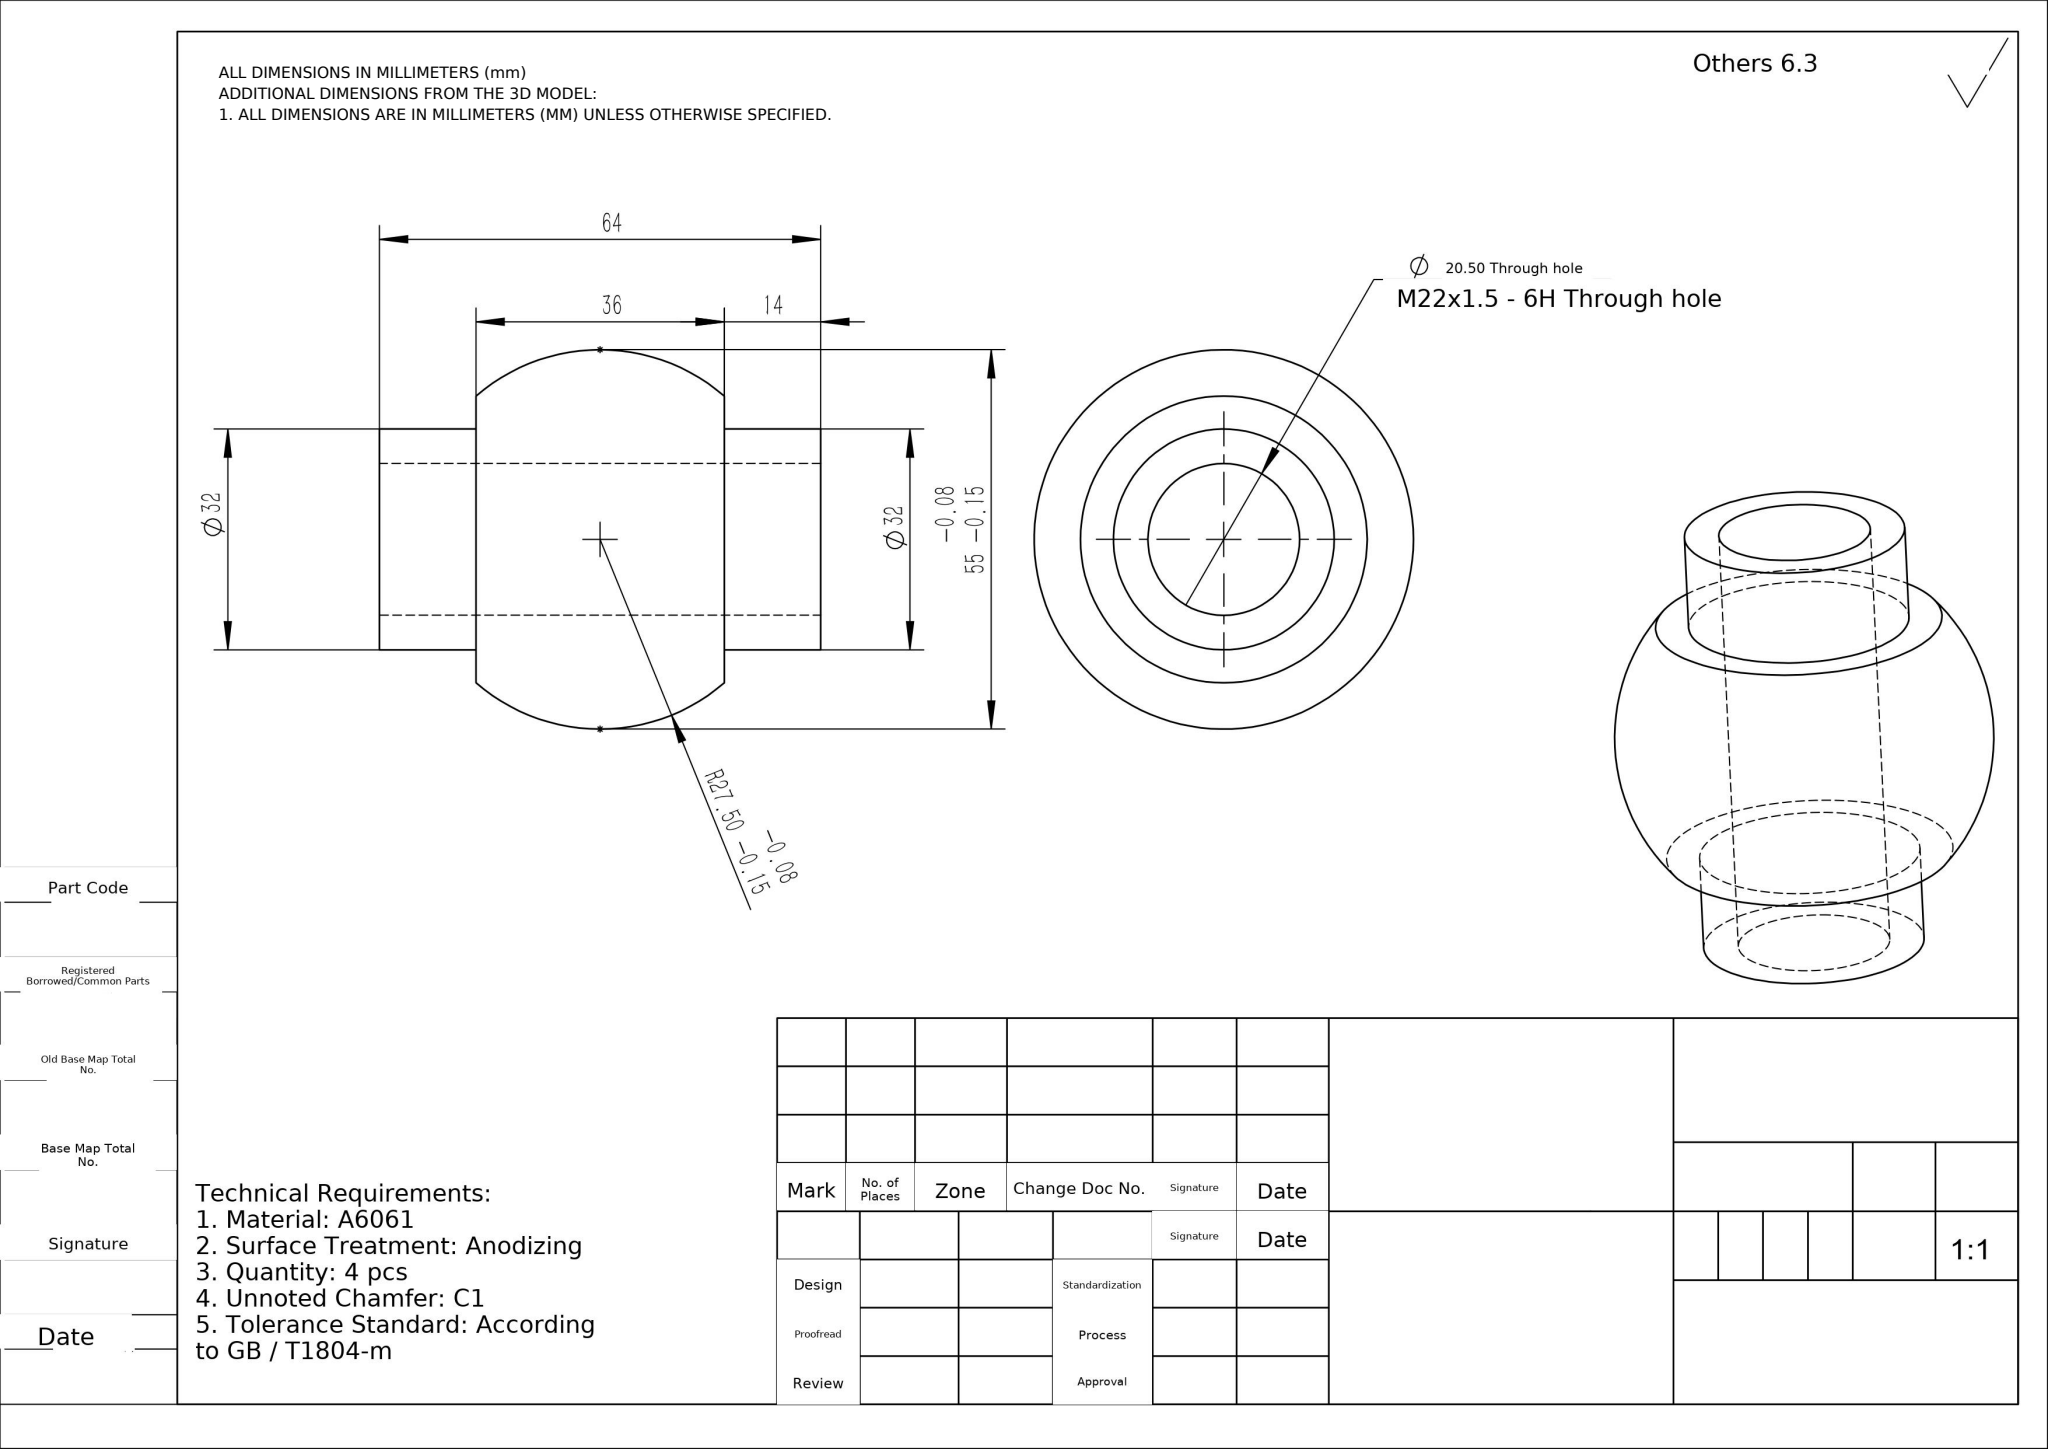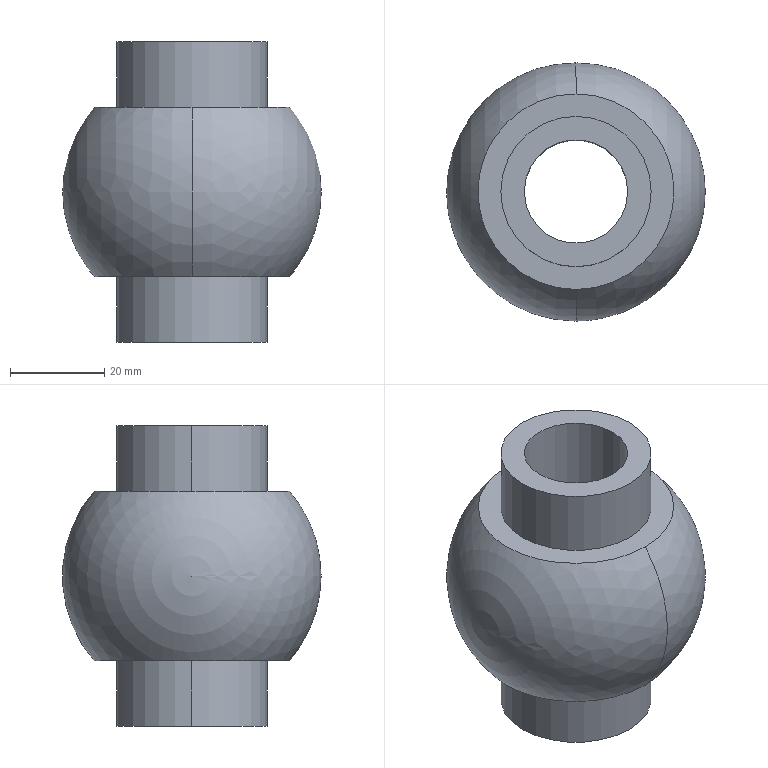Part | NX | mm | Spherical Flanged Bushing | 1 solid | 12 faces | box 55 x 55 x 64 mm | volume 71506 mm3 | cylinder 6 | plane 4 | sphere 2 | commonest cylinder face diameters 32 x4 22 x2
STEP:
#1=COLOUR_RGB('',0.,0.502,0.502);
#2=FILL_AREA_STYLE_COLOUR('',#1);
#3=FILL_AREA_STYLE('',(#2));
#4=SURFACE_STYLE_FILL_AREA(#3);
#5=SURFACE_SIDE_STYLE('',(#4));
#6=SURFACE_STYLE_USAGE(.BOTH.,#5);
#7=PRESENTATION_STYLE_ASSIGNMENT((#6));
#8=CARTESIAN_POINT('',(-11.,0.,-32.));
#9=VERTEX_POINT('',#8);
#10=CARTESIAN_POINT('',(11.,0.,-32.));
#11=VERTEX_POINT('',#10);
#12=CARTESIAN_POINT('',(0.,0.,-32.));
#13=DIRECTION('',(0.,0.,1.));
#14=DIRECTION('',(1.,0.,0.));
#15=AXIS2_PLACEMENT_3D('',#12,#13,#14);
#16=CIRCLE('',#15,11.);
#17=EDGE_CURVE('',#9,#11,#16,.T.);
#18=ORIENTED_EDGE('',*,*,#17,.F.);
#19=CARTESIAN_POINT('',(-11.,0.,32.));
#20=VERTEX_POINT('',#19);
#21=CARTESIAN_POINT('',(-11.,0.,32.));
#22=DIRECTION('',(0.,0.,1.));
#23=VECTOR('',#22,1000.);
#24=LINE('',#21,#23);
#25=EDGE_CURVE('',#9,#20,#24,.T.);
#26=ORIENTED_EDGE('',*,*,#25,.T.);
#27=CARTESIAN_POINT('',(11.,0.,32.));
#28=VERTEX_POINT('',#27);
#29=CARTESIAN_POINT('',(0.,0.,32.));
#30=DIRECTION('',(0.,0.,1.));
#31=DIRECTION('',(1.,0.,0.));
#32=AXIS2_PLACEMENT_3D('',#29,#30,#31);
#33=CIRCLE('',#32,11.);
#34=EDGE_CURVE('',#20,#28,#33,.T.);
#35=ORIENTED_EDGE('',*,*,#34,.T.);
#36=CARTESIAN_POINT('',(11.,0.,32.));
#37=DIRECTION('',(0.,0.,1.));
#38=VECTOR('',#37,1000.);
#39=LINE('',#36,#38);
#40=EDGE_CURVE('',#11,#28,#39,.T.);
#41=ORIENTED_EDGE('',*,*,#40,.F.);
#42=EDGE_LOOP('',(#18,#26,#35,#41));
#43=FACE_OUTER_BOUND('',#42,.T.);
#44=CARTESIAN_POINT('',(0.,0.,32.));
#45=DIRECTION('',(0.,0.,1.));
#46=DIRECTION('',(1.,0.,0.));
#47=AXIS2_PLACEMENT_3D('',#44,#45,#46);
#48=CYLINDRICAL_SURFACE('',#47,11.);
#49=ADVANCED_FACE('',(#43),#48,.F.);
#50=CARTESIAN_POINT('',(16.,0.,32.));
#51=VERTEX_POINT('',#50);
#52=CARTESIAN_POINT('',(-16.,0.,32.));
#53=VERTEX_POINT('',#52);
#54=CARTESIAN_POINT('',(0.,0.,32.));
#55=DIRECTION('',(0.,0.,1.));
#56=DIRECTION('',(1.,0.,0.));
#57=AXIS2_PLACEMENT_3D('',#54,#55,#56);
#58=CIRCLE('',#57,16.);
#59=EDGE_CURVE('',#51,#53,#58,.T.);
#60=ORIENTED_EDGE('',*,*,#59,.F.);
#61=CARTESIAN_POINT('',(16.,0.,18.));
#62=VERTEX_POINT('',#61);
#63=CARTESIAN_POINT('',(16.,0.,32.));
#64=DIRECTION('',(0.,0.,-1.));
#65=VECTOR('',#64,1000.);
#66=LINE('',#63,#65);
#67=EDGE_CURVE('',#51,#62,#66,.T.);
#68=ORIENTED_EDGE('',*,*,#67,.T.);
#69=CARTESIAN_POINT('',(-16.,0.,18.));
#70=VERTEX_POINT('',#69);
#71=CARTESIAN_POINT('',(0.,0.,18.));
#72=DIRECTION('',(0.,0.,-1.));
#73=DIRECTION('',(-1.,0.,0.));
#74=AXIS2_PLACEMENT_3D('',#71,#72,#73);
#75=CIRCLE('',#74,16.);
#76=EDGE_CURVE('',#70,#62,#75,.T.);
#77=ORIENTED_EDGE('',*,*,#76,.F.);
#78=CARTESIAN_POINT('',(-16.,0.,32.));
#79=DIRECTION('',(0.,0.,-1.));
#80=VECTOR('',#79,1000.);
#81=LINE('',#78,#80);
#82=EDGE_CURVE('',#53,#70,#81,.T.);
#83=ORIENTED_EDGE('',*,*,#82,.F.);
#84=EDGE_LOOP('',(#60,#68,#77,#83));
#85=FACE_OUTER_BOUND('',#84,.T.);
#86=CARTESIAN_POINT('',(0.,0.,32.));
#87=DIRECTION('',(0.,0.,-1.));
#88=DIRECTION('',(-1.,0.,0.));
#89=AXIS2_PLACEMENT_3D('',#86,#87,#88);
#90=CYLINDRICAL_SURFACE('',#89,16.);
#91=ADVANCED_FACE('',(#85),#90,.T.);
#92=CARTESIAN_POINT('',(0.,-20.791,18.));
#93=VERTEX_POINT('',#92);
#94=CARTESIAN_POINT('',(-0.,20.791,18.));
#95=VERTEX_POINT('',#94);
#96=CARTESIAN_POINT('',(0.,0.,18.));
#97=DIRECTION('',(0.,0.,-1.));
#98=DIRECTION('',(-1.,0.,0.));
#99=AXIS2_PLACEMENT_3D('',#96,#97,#98);
#100=CIRCLE('',#99,20.791);
#101=EDGE_CURVE('',#93,#95,#100,.T.);
#102=ORIENTED_EDGE('',*,*,#101,.T.);
#103=CARTESIAN_POINT('',(-0.,20.791,-18.));
#104=VERTEX_POINT('',#103);
#105=CARTESIAN_POINT('',(0.,0.,0.));
#106=DIRECTION('',(-1.,-0.,0.));
#107=DIRECTION('',(0.,-1.,0.));
#108=AXIS2_PLACEMENT_3D('',#105,#106,#107);
#109=CIRCLE('',#108,27.5);
#110=EDGE_CURVE('',#95,#104,#109,.T.);
#111=ORIENTED_EDGE('',*,*,#110,.T.);
#112=CARTESIAN_POINT('',(0.,-20.791,-18.));
#113=VERTEX_POINT('',#112);
#114=CARTESIAN_POINT('',(0.,0.,-18.));
#115=DIRECTION('',(0.,0.,-1.));
#116=DIRECTION('',(-1.,0.,0.));
#117=AXIS2_PLACEMENT_3D('',#114,#115,#116);
#118=CIRCLE('',#117,20.791);
#119=EDGE_CURVE('',#113,#104,#118,.T.);
#120=ORIENTED_EDGE('',*,*,#119,.F.);
#121=CARTESIAN_POINT('',(0.,0.,0.));
#122=DIRECTION('',(1.,0.,0.));
#123=DIRECTION('',(0.,0.,-1.));
#124=AXIS2_PLACEMENT_3D('',#121,#122,#123);
#125=CIRCLE('',#124,27.5);
#126=EDGE_CURVE('',#93,#113,#125,.T.);
#127=ORIENTED_EDGE('',*,*,#126,.F.);
#128=EDGE_LOOP('',(#102,#111,#120,#127));
#129=FACE_OUTER_BOUND('',#128,.T.);
#130=CARTESIAN_POINT('',(0.,0.,0.));
#131=DIRECTION('',(-1.,0.,0.));
#132=DIRECTION('',(0.,-1.,0.));
#133=AXIS2_PLACEMENT_3D('',#130,#131,#132);
#134=SPHERICAL_SURFACE('',#133,27.5);
#135=ADVANCED_FACE('',(#129),#134,.T.);
#136=CARTESIAN_POINT('',(16.,0.,-18.));
#137=VERTEX_POINT('',#136);
#138=CARTESIAN_POINT('',(-16.,0.,-18.));
#139=VERTEX_POINT('',#138);
#140=CARTESIAN_POINT('',(0.,0.,-18.));
#141=DIRECTION('',(0.,0.,1.));
#142=DIRECTION('',(1.,0.,0.));
#143=AXIS2_PLACEMENT_3D('',#140,#141,#142);
#144=CIRCLE('',#143,16.);
#145=EDGE_CURVE('',#137,#139,#144,.T.);
#146=ORIENTED_EDGE('',*,*,#145,.F.);
#147=CARTESIAN_POINT('',(16.,0.,-32.));
#148=VERTEX_POINT('',#147);
#149=CARTESIAN_POINT('',(16.,0.,32.));
#150=DIRECTION('',(0.,0.,-1.));
#151=VECTOR('',#150,1000.);
#152=LINE('',#149,#151);
#153=EDGE_CURVE('',#137,#148,#152,.T.);
#154=ORIENTED_EDGE('',*,*,#153,.T.);
#155=CARTESIAN_POINT('',(-16.,0.,-32.));
#156=VERTEX_POINT('',#155);
#157=CARTESIAN_POINT('',(0.,0.,-32.));
#158=DIRECTION('',(0.,0.,1.));
#159=DIRECTION('',(1.,0.,0.));
#160=AXIS2_PLACEMENT_3D('',#157,#158,#159);
#161=CIRCLE('',#160,16.);
#162=EDGE_CURVE('',#148,#156,#161,.T.);
#163=ORIENTED_EDGE('',*,*,#162,.T.);
#164=CARTESIAN_POINT('',(-16.,0.,32.));
#165=DIRECTION('',(0.,0.,-1.));
#166=VECTOR('',#165,1000.);
#167=LINE('',#164,#166);
#168=EDGE_CURVE('',#139,#156,#167,.T.);
#169=ORIENTED_EDGE('',*,*,#168,.F.);
#170=EDGE_LOOP('',(#146,#154,#163,#169));
#171=FACE_OUTER_BOUND('',#170,.T.);
#172=CARTESIAN_POINT('',(0.,0.,32.));
#173=DIRECTION('',(0.,0.,-1.));
#174=DIRECTION('',(-1.,0.,0.));
#175=AXIS2_PLACEMENT_3D('',#172,#173,#174);
#176=CYLINDRICAL_SURFACE('',#175,16.);
#177=ADVANCED_FACE('',(#171),#176,.T.);
#178=ORIENTED_EDGE('',*,*,#153,.F.);
#179=CARTESIAN_POINT('',(0.,0.,-18.));
#180=DIRECTION('',(0.,0.,1.));
#181=DIRECTION('',(1.,0.,0.));
#182=AXIS2_PLACEMENT_3D('',#179,#180,#181);
#183=CIRCLE('',#182,16.);
#184=EDGE_CURVE('',#139,#137,#183,.T.);
#185=ORIENTED_EDGE('',*,*,#184,.F.);
#186=ORIENTED_EDGE('',*,*,#168,.T.);
#187=CARTESIAN_POINT('',(0.,0.,-32.));
#188=DIRECTION('',(0.,0.,1.));
#189=DIRECTION('',(1.,0.,0.));
#190=AXIS2_PLACEMENT_3D('',#187,#188,#189);
#191=CIRCLE('',#190,16.);
#192=EDGE_CURVE('',#156,#148,#191,.T.);
#193=ORIENTED_EDGE('',*,*,#192,.T.);
#194=EDGE_LOOP('',(#178,#185,#186,#193));
#195=FACE_OUTER_BOUND('',#194,.T.);
#196=CARTESIAN_POINT('',(0.,0.,32.));
#197=DIRECTION('',(0.,0.,-1.));
#198=DIRECTION('',(-1.,0.,0.));
#199=AXIS2_PLACEMENT_3D('',#196,#197,#198);
#200=CYLINDRICAL_SURFACE('',#199,16.);
#201=ADVANCED_FACE('',(#195),#200,.T.);
#202=CARTESIAN_POINT('',(0.,0.,-32.));
#203=DIRECTION('',(0.,0.,1.));
#204=DIRECTION('',(1.,0.,0.));
#205=AXIS2_PLACEMENT_3D('',#202,#203,#204);
#206=CIRCLE('',#205,11.);
#207=EDGE_CURVE('',#11,#9,#206,.T.);
#208=ORIENTED_EDGE('',*,*,#207,.T.);
#209=ORIENTED_EDGE('',*,*,#17,.T.);
#210=EDGE_LOOP('',(#208,#209));
#211=FACE_BOUND('',#210,.T.);
#212=ORIENTED_EDGE('',*,*,#192,.F.);
#213=ORIENTED_EDGE('',*,*,#162,.F.);
#214=EDGE_LOOP('',(#212,#213));
#215=FACE_OUTER_BOUND('',#214,.T.);
#216=CARTESIAN_POINT('',(0.,0.,-32.));
#217=DIRECTION('',(0.,0.,1.));
#218=DIRECTION('',(1.,0.,0.));
#219=AXIS2_PLACEMENT_3D('',#216,#217,#218);
#220=PLANE('',#219);
#221=ADVANCED_FACE('',(#211,#215),#220,.F.);
#222=ORIENTED_EDGE('',*,*,#119,.T.);
#223=CARTESIAN_POINT('',(0.,0.,-18.));
#224=DIRECTION('',(0.,0.,-1.));
#225=DIRECTION('',(-1.,0.,0.));
#226=AXIS2_PLACEMENT_3D('',#223,#224,#225);
#227=CIRCLE('',#226,20.791);
#228=EDGE_CURVE('',#104,#113,#227,.T.);
#229=ORIENTED_EDGE('',*,*,#228,.T.);
#230=EDGE_LOOP('',(#222,#229));
#231=FACE_OUTER_BOUND('',#230,.T.);
#232=ORIENTED_EDGE('',*,*,#184,.T.);
#233=ORIENTED_EDGE('',*,*,#145,.T.);
#234=EDGE_LOOP('',(#232,#233));
#235=FACE_BOUND('',#234,.T.);
#236=CARTESIAN_POINT('',(0.,0.,-18.));
#237=DIRECTION('',(0.,0.,1.));
#238=DIRECTION('',(1.,0.,0.));
#239=AXIS2_PLACEMENT_3D('',#236,#237,#238);
#240=PLANE('',#239);
#241=ADVANCED_FACE('',(#231,#235),#240,.F.);
#242=ORIENTED_EDGE('',*,*,#101,.F.);
#243=CARTESIAN_POINT('',(0.,0.,18.));
#244=DIRECTION('',(0.,0.,-1.));
#245=DIRECTION('',(-1.,0.,0.));
#246=AXIS2_PLACEMENT_3D('',#243,#244,#245);
#247=CIRCLE('',#246,20.791);
#248=EDGE_CURVE('',#95,#93,#247,.T.);
#249=ORIENTED_EDGE('',*,*,#248,.F.);
#250=EDGE_LOOP('',(#242,#249));
#251=FACE_OUTER_BOUND('',#250,.T.);
#252=ORIENTED_EDGE('',*,*,#76,.T.);
#253=CARTESIAN_POINT('',(0.,0.,18.));
#254=DIRECTION('',(0.,0.,-1.));
#255=DIRECTION('',(-1.,0.,0.));
#256=AXIS2_PLACEMENT_3D('',#253,#254,#255);
#257=CIRCLE('',#256,16.);
#258=EDGE_CURVE('',#62,#70,#257,.T.);
#259=ORIENTED_EDGE('',*,*,#258,.T.);
#260=EDGE_LOOP('',(#252,#259));
#261=FACE_BOUND('',#260,.T.);
#262=CARTESIAN_POINT('',(0.,0.,18.));
#263=DIRECTION('',(0.,0.,-1.));
#264=DIRECTION('',(-1.,0.,0.));
#265=AXIS2_PLACEMENT_3D('',#262,#263,#264);
#266=PLANE('',#265);
#267=ADVANCED_FACE('',(#251,#261),#266,.F.);
#268=ORIENTED_EDGE('',*,*,#110,.F.);
#269=ORIENTED_EDGE('',*,*,#248,.T.);
#270=ORIENTED_EDGE('',*,*,#126,.T.);
#271=ORIENTED_EDGE('',*,*,#228,.F.);
#272=EDGE_LOOP('',(#268,#269,#270,#271));
#273=FACE_OUTER_BOUND('',#272,.T.);
#274=CARTESIAN_POINT('',(0.,0.,0.));
#275=DIRECTION('',(-1.,0.,0.));
#276=DIRECTION('',(0.,-1.,0.));
#277=AXIS2_PLACEMENT_3D('',#274,#275,#276);
#278=SPHERICAL_SURFACE('',#277,27.5);
#279=ADVANCED_FACE('',(#273),#278,.T.);
#280=CARTESIAN_POINT('',(0.,0.,32.));
#281=DIRECTION('',(0.,0.,1.));
#282=DIRECTION('',(1.,0.,0.));
#283=AXIS2_PLACEMENT_3D('',#280,#281,#282);
#284=CIRCLE('',#283,11.);
#285=EDGE_CURVE('',#28,#20,#284,.T.);
#286=ORIENTED_EDGE('',*,*,#285,.F.);
#287=ORIENTED_EDGE('',*,*,#34,.F.);
#288=EDGE_LOOP('',(#286,#287));
#289=FACE_BOUND('',#288,.T.);
#290=CARTESIAN_POINT('',(0.,0.,32.));
#291=DIRECTION('',(0.,0.,1.));
#292=DIRECTION('',(1.,0.,0.));
#293=AXIS2_PLACEMENT_3D('',#290,#291,#292);
#294=CIRCLE('',#293,16.);
#295=EDGE_CURVE('',#53,#51,#294,.T.);
#296=ORIENTED_EDGE('',*,*,#295,.T.);
#297=ORIENTED_EDGE('',*,*,#59,.T.);
#298=EDGE_LOOP('',(#296,#297));
#299=FACE_OUTER_BOUND('',#298,.T.);
#300=CARTESIAN_POINT('',(0.,0.,32.));
#301=DIRECTION('',(0.,0.,1.));
#302=DIRECTION('',(1.,0.,0.));
#303=AXIS2_PLACEMENT_3D('',#300,#301,#302);
#304=PLANE('',#303);
#305=ADVANCED_FACE('',(#289,#299),#304,.T.);
#306=ORIENTED_EDGE('',*,*,#67,.F.);
#307=ORIENTED_EDGE('',*,*,#295,.F.);
#308=ORIENTED_EDGE('',*,*,#82,.T.);
#309=ORIENTED_EDGE('',*,*,#258,.F.);
#310=EDGE_LOOP('',(#306,#307,#308,#309));
#311=FACE_OUTER_BOUND('',#310,.T.);
#312=CARTESIAN_POINT('',(0.,0.,32.));
#313=DIRECTION('',(0.,0.,-1.));
#314=DIRECTION('',(-1.,0.,0.));
#315=AXIS2_PLACEMENT_3D('',#312,#313,#314);
#316=CYLINDRICAL_SURFACE('',#315,16.);
#317=ADVANCED_FACE('',(#311),#316,.T.);
#318=ORIENTED_EDGE('',*,*,#25,.F.);
#319=ORIENTED_EDGE('',*,*,#207,.F.);
#320=ORIENTED_EDGE('',*,*,#40,.T.);
#321=ORIENTED_EDGE('',*,*,#285,.T.);
#322=EDGE_LOOP('',(#318,#319,#320,#321));
#323=FACE_OUTER_BOUND('',#322,.T.);
#324=CARTESIAN_POINT('',(0.,0.,32.));
#325=DIRECTION('',(0.,0.,1.));
#326=DIRECTION('',(1.,0.,0.));
#327=AXIS2_PLACEMENT_3D('',#324,#325,#326);
#328=CYLINDRICAL_SURFACE('',#327,11.);
#329=ADVANCED_FACE('',(#323),#328,.F.);
#330=CLOSED_SHELL('',(#49,#91,#135,#177,#201,#221,#241,#267,#279,#305,#317,#329));
#331=MANIFOLD_SOLID_BREP('',#330);
#332=CARTESIAN_POINT('',(0.,0.,0.));
#333=DIRECTION('',(0.,0.,1.));
#334=DIRECTION('',(1.,0.,0.));
#335=AXIS2_PLACEMENT_3D('',#332,#333,#334);
#336=(LENGTH_UNIT()NAMED_UNIT(*)SI_UNIT(.MILLI.,.METRE.));
#337=UNCERTAINTY_MEASURE_WITH_UNIT(LENGTH_MEASURE(0.00001),#336,'','');
#338=(NAMED_UNIT(*)PLANE_ANGLE_UNIT()SI_UNIT($,.RADIAN.));
#339=(NAMED_UNIT(*)SI_UNIT($,.STERADIAN.)SOLID_ANGLE_UNIT());
#340=(GEOMETRIC_REPRESENTATION_CONTEXT(3)GLOBAL_UNCERTAINTY_ASSIGNED_CONTEXT((#337))GLOBAL_UNIT_ASSIGNED_CONTEXT((#336,#338,#339))REPRESENTATION_CONTEXT('',''));
#341=ADVANCED_BREP_SHAPE_REPRESENTATION('',(#331,#335),#340);
#342=STYLED_ITEM('',(#7),#341);
#343=PRESENTATION_LAYER_ASSIGNMENT('','',(#342));
#344=COLOUR_RGB('',0.,0.502,0.502);
#345=FILL_AREA_STYLE_COLOUR('',#344);
#346=FILL_AREA_STYLE('',(#345));
#347=SURFACE_STYLE_FILL_AREA(#346);
#348=SURFACE_SIDE_STYLE('',(#347));
#349=SURFACE_STYLE_USAGE(.BOTH.,#348);
#350=PRESENTATION_STYLE_ASSIGNMENT((#349));
#351=STYLED_ITEM('',(#350),#331);
#352=PRESENTATION_LAYER_ASSIGNMENT('','',(#351));
#353=(LENGTH_UNIT()NAMED_UNIT(*)SI_UNIT(.MILLI.,.METRE.));
#354=UNCERTAINTY_MEASURE_WITH_UNIT(LENGTH_MEASURE(0.00001),#353,'','');
#355=(NAMED_UNIT(*)PLANE_ANGLE_UNIT()SI_UNIT($,.RADIAN.));
#356=(NAMED_UNIT(*)SI_UNIT($,.STERADIAN.)SOLID_ANGLE_UNIT());
#357=(GEOMETRIC_REPRESENTATION_CONTEXT(3)GLOBAL_UNCERTAINTY_ASSIGNED_CONTEXT((#354))GLOBAL_UNIT_ASSIGNED_CONTEXT((#353,#355,#356))REPRESENTATION_CONTEXT('',''));
#358=MECHANICAL_DESIGN_GEOMETRIC_PRESENTATION_REPRESENTATION('',(#351),#357);
#359=(LENGTH_UNIT()NAMED_UNIT(*)SI_UNIT(.MILLI.,.METRE.));
#360=UNCERTAINTY_MEASURE_WITH_UNIT(LENGTH_MEASURE(0.00001),#359,'','');
#361=(NAMED_UNIT(*)PLANE_ANGLE_UNIT()SI_UNIT($,.RADIAN.));
#362=(NAMED_UNIT(*)SI_UNIT($,.STERADIAN.)SOLID_ANGLE_UNIT());
#363=(GEOMETRIC_REPRESENTATION_CONTEXT(3)GLOBAL_UNCERTAINTY_ASSIGNED_CONTEXT((#360))GLOBAL_UNIT_ASSIGNED_CONTEXT((#359,#361,#362))REPRESENTATION_CONTEXT('',''));
#364=MECHANICAL_DESIGN_GEOMETRIC_PRESENTATION_REPRESENTATION('',(#342),#363);